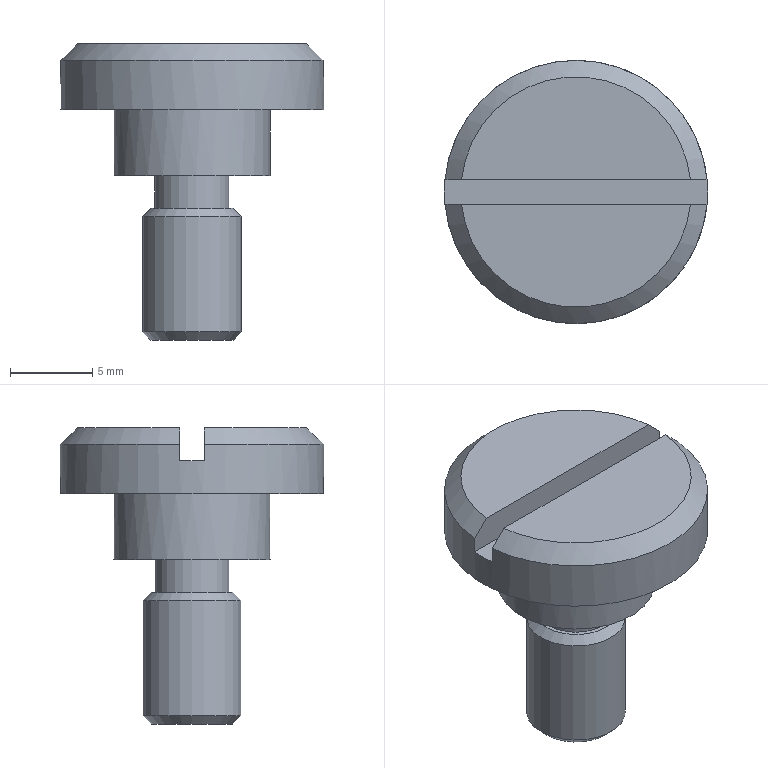Component | NX | DRILL_BUSH_SCREW | 1 solid | 17 faces | volume 1271 mm3 | plane 9 | cylinder 4 | cone 4 | commonest cylinder face diameters 6 x1 4.5 x1 9.5 x1 16 x1